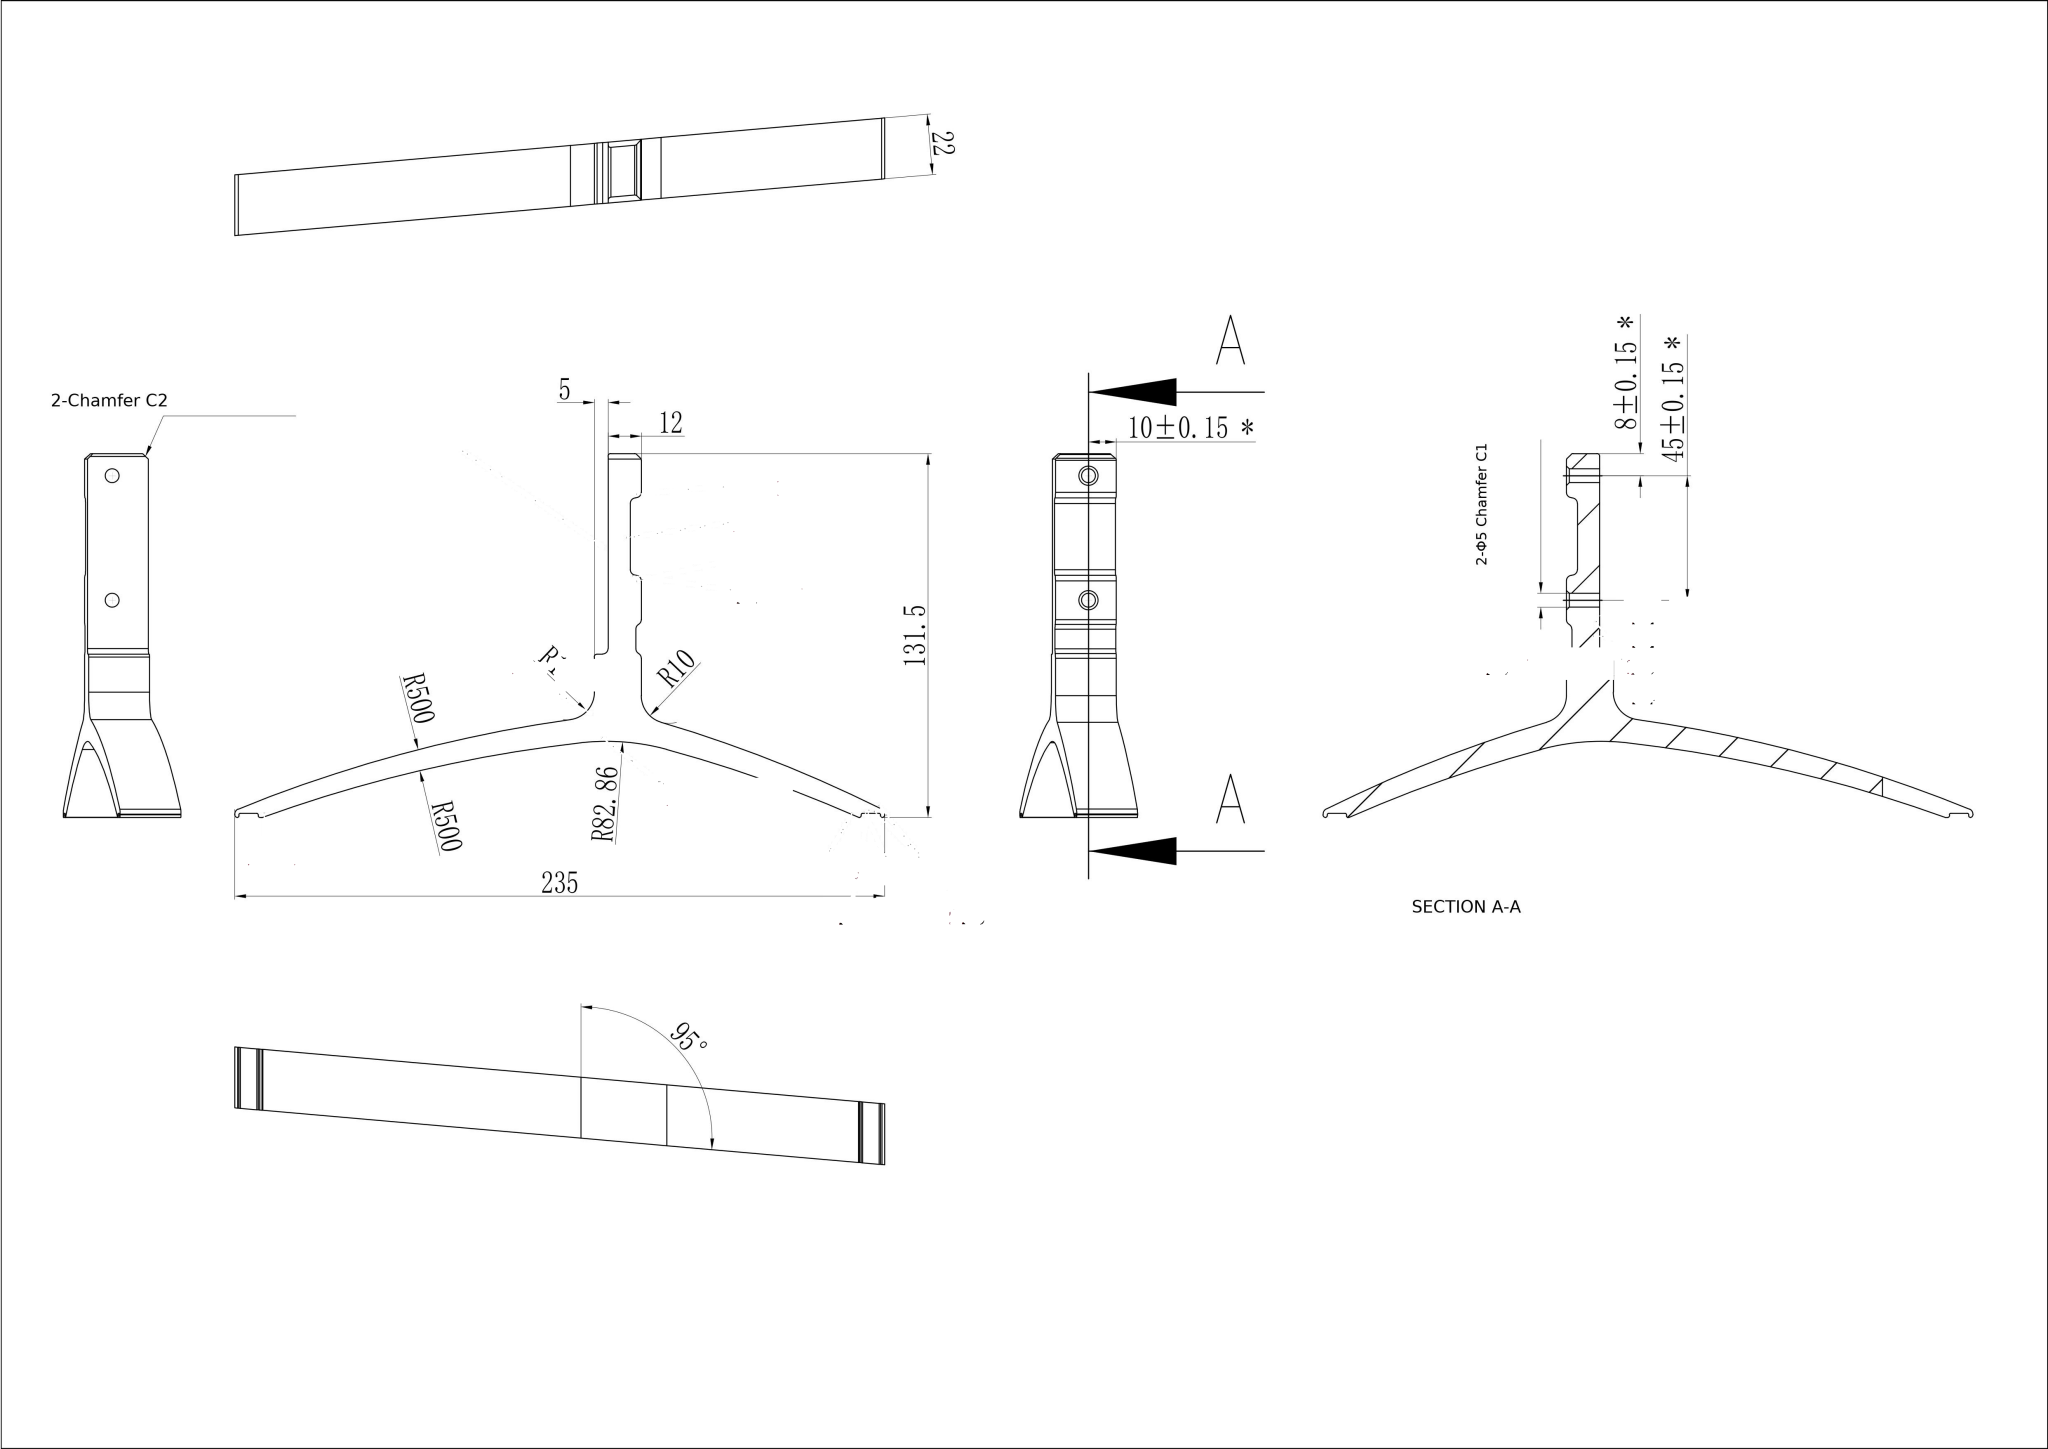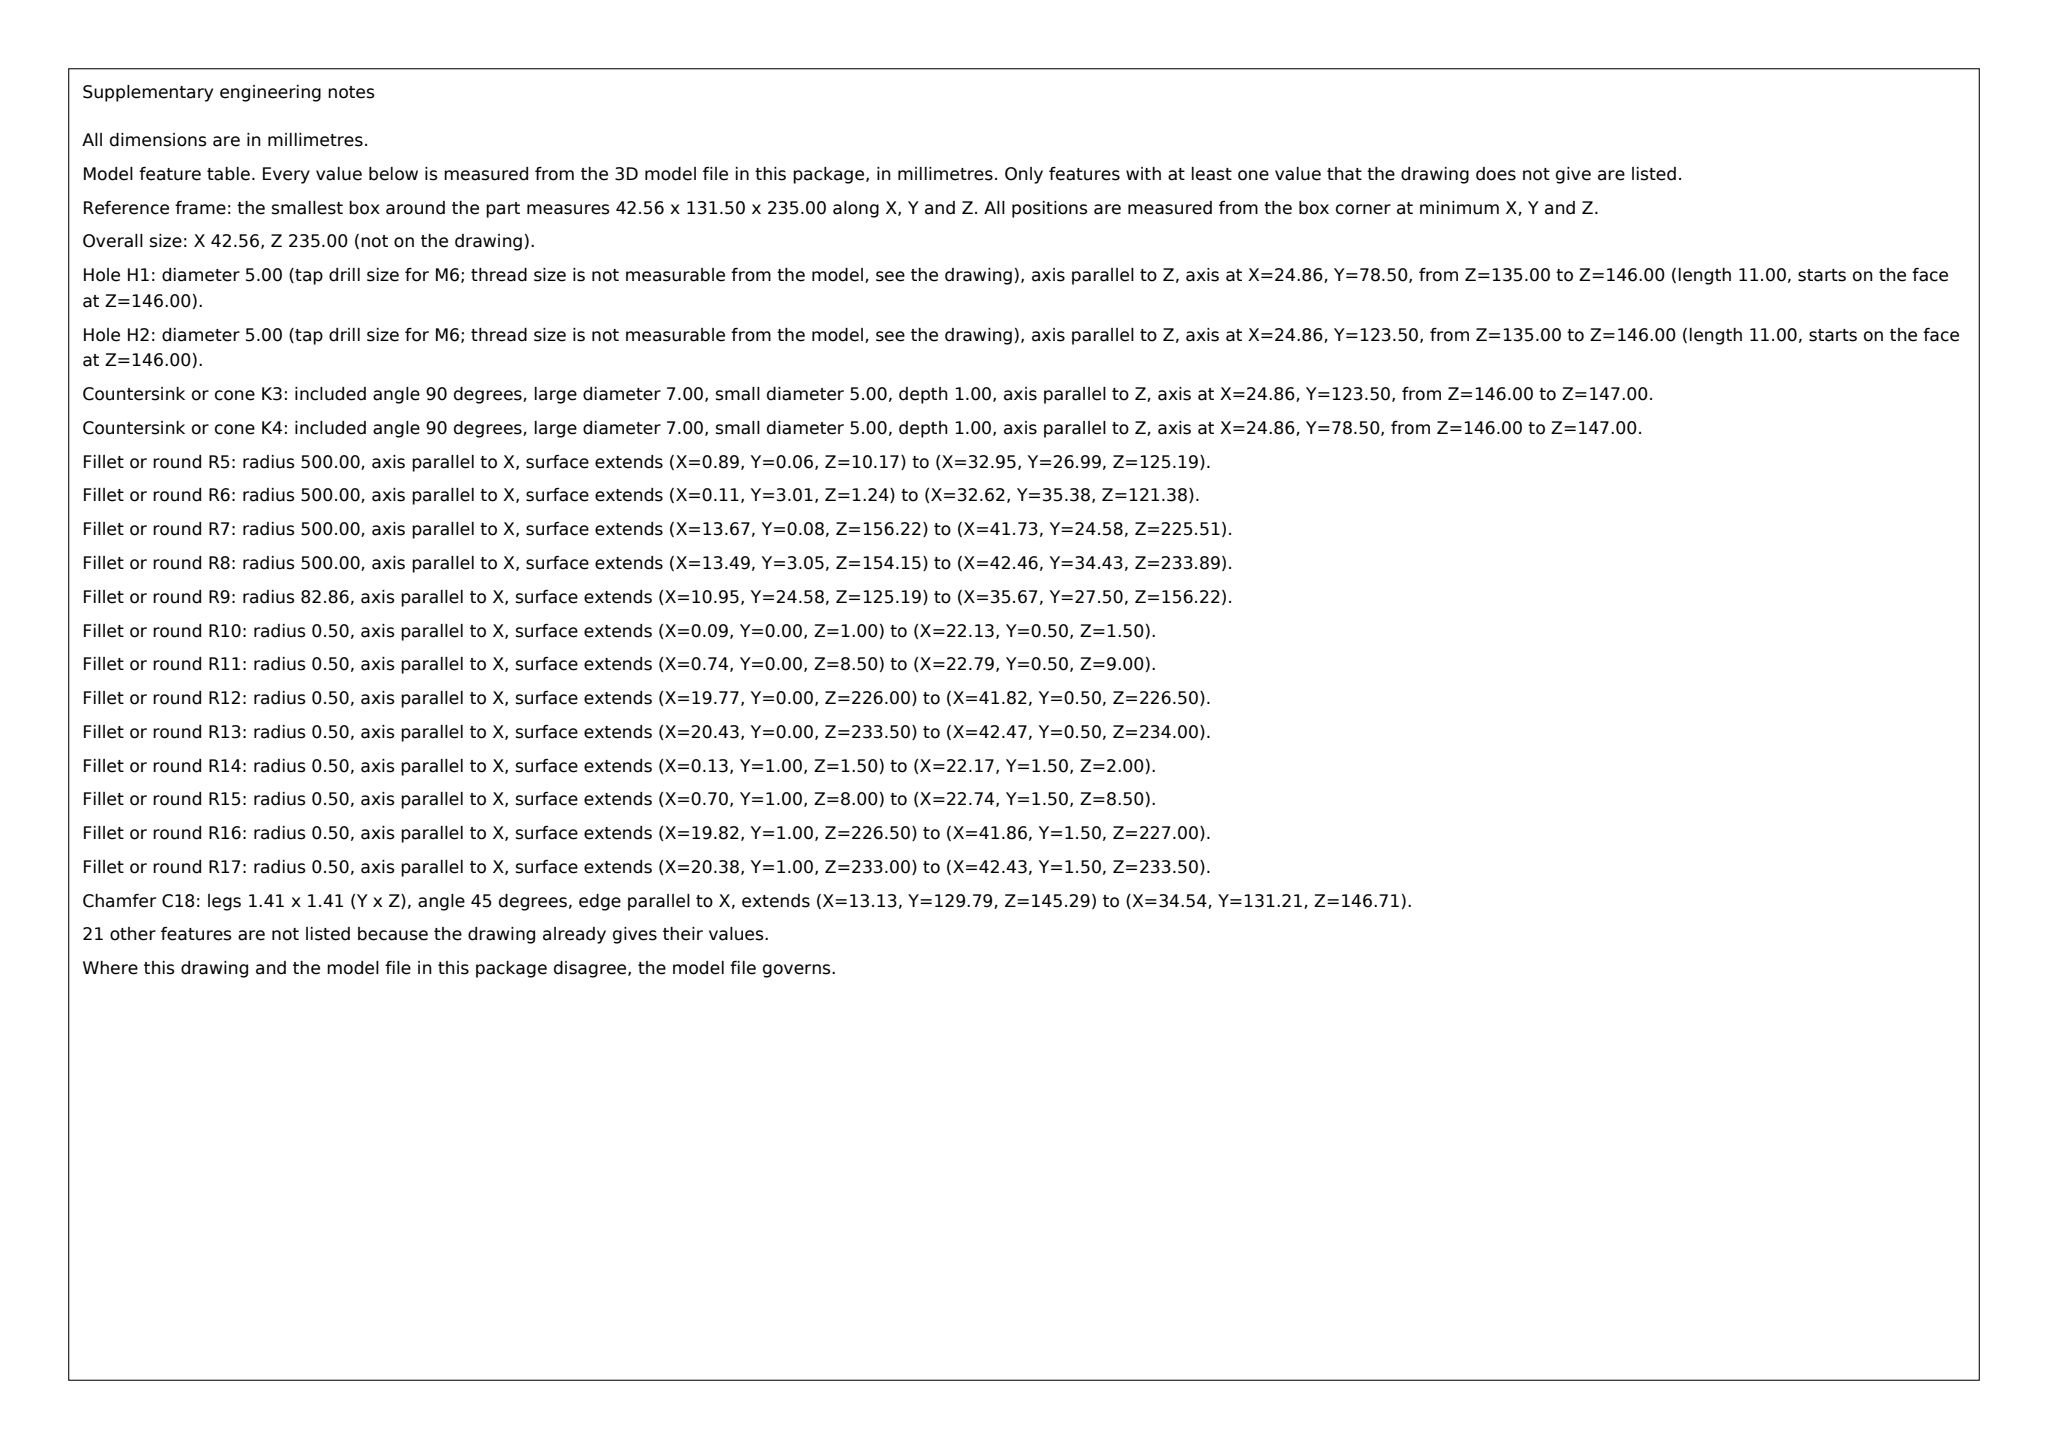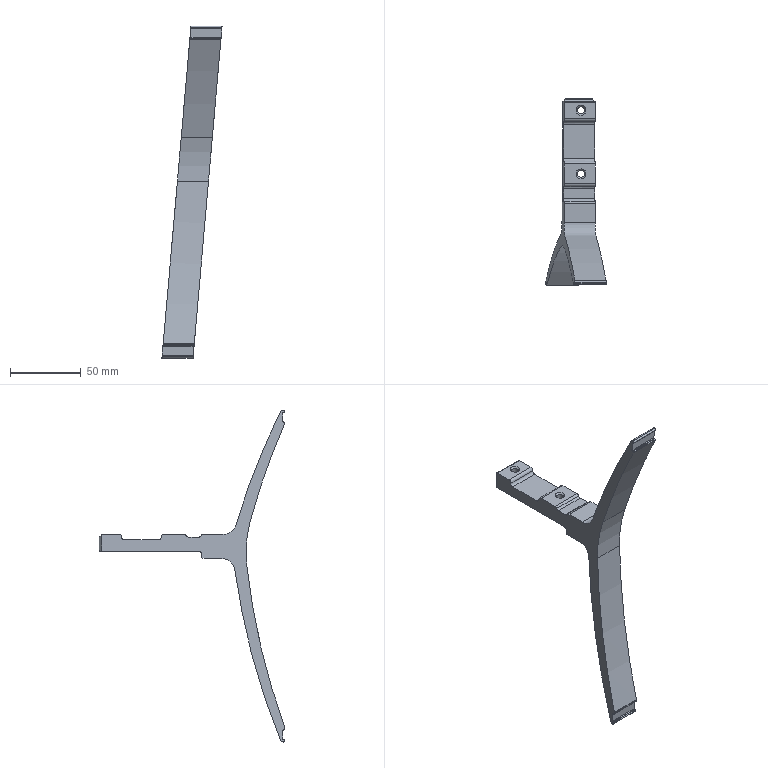Part | SolidWorks | mm | 1 solid | 66 faces | box 42.56 x 131.5 x 235 mm | volume 64539 mm3 | cylinder 38 | plane 24 | cone 4 | commonest cylinder face diameters 4 x11 2 x8 1 x8 5 x4 1000 x4 20 x2 165.711 x1